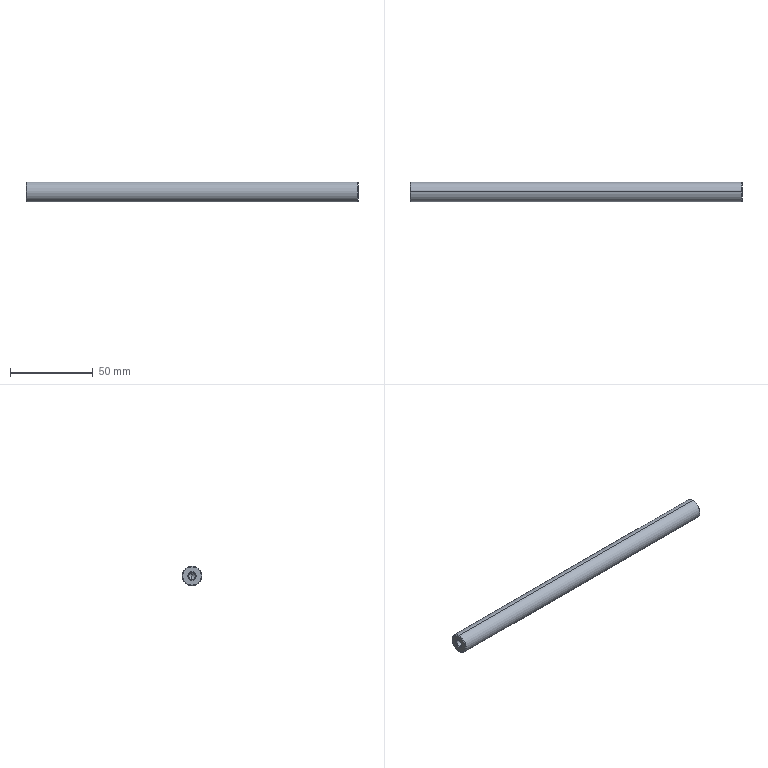Component | SolidWorks | D12-200-1 | 1 solid | 20 faces | box 200 x 12 x 12 mm | volume 22253 mm3 | cone 12 | cylinder 6 | plane 2 | commonest cylinder face diameters 4.2 x4 12 x2
build123d program:
from build123d import *

# Parameters (mm, degrees)
SKETCH1_R                   = 6
BOSS_EXTRUDE1_DEPTH         = 200
CHAMFER1_SIZE               = 0.5
M5_TAPPED_HOLE1_D           = 4.2
M5_TAPPED_HOLE1_DEPTH       = 12.4
M5_TAPPED_HOLE1_CSINK_D     = 5.05
M5_TAPPED_HOLE1_CSINK_ANGLE = 90
M5_TAPPED_HOLE1_TIP         = 1.262
M5_TAPPED_HOLE2_D           = 4.2
M5_TAPPED_HOLE2_DEPTH       = 12.4
M5_TAPPED_HOLE2_CSINK_D     = 5.05
M5_TAPPED_HOLE2_CSINK_ANGLE = 90
M5_TAPPED_HOLE2_TIP         = 1.262


with BuildPart() as part:
    # Sketch1 → Boss-Extrude1 (new body)
    with BuildSketch(Plane.XY):
        with Locations((-21.5, 75)):
            Circle(SKETCH1_R)
    extrude(amount=BOSS_EXTRUDE1_DEPTH)

    # Chamfer1
    chamfer1_edges = [part.edges().sort_by_distance(p)[0] for p in [
        (-27.5, 75, 0),
        (-27.5, 75, 200),
    ]]
    chamfer(chamfer1_edges, length=CHAMFER1_SIZE)

    # M5 Tapped Hole1
    with Locations(Plane(origin=(0, 0, 0), x_dir=(-1, 0, 0), z_dir=(0, 0, -1))):
        with Locations((21.5, 75)):
            CounterSinkHole(M5_TAPPED_HOLE1_D / 2, M5_TAPPED_HOLE1_CSINK_D / 2, depth=M5_TAPPED_HOLE1_DEPTH, counter_sink_angle=M5_TAPPED_HOLE1_CSINK_ANGLE)
            with Locations((0, 0, -(M5_TAPPED_HOLE1_DEPTH + M5_TAPPED_HOLE1_TIP / 2))):  # 118° drill point
                Cone(0, M5_TAPPED_HOLE1_D / 2, M5_TAPPED_HOLE1_TIP, mode=Mode.SUBTRACT)

    # M5 Tapped Hole2
    with Locations(Plane.XY.offset(200)):
        with Locations((-21.5, 75)):
            CounterSinkHole(M5_TAPPED_HOLE2_D / 2, M5_TAPPED_HOLE2_CSINK_D / 2, depth=M5_TAPPED_HOLE2_DEPTH, counter_sink_angle=M5_TAPPED_HOLE2_CSINK_ANGLE)
            with Locations((0, 0, -(M5_TAPPED_HOLE2_DEPTH + M5_TAPPED_HOLE2_TIP / 2))):  # 118° drill point
                Cone(0, M5_TAPPED_HOLE2_D / 2, M5_TAPPED_HOLE2_TIP, mode=Mode.SUBTRACT)


solid = part.part

# Placed as in the assembly
solid = solid.moved(Location((-170.981, -6.484, 35.5), (0, 90, 0)))